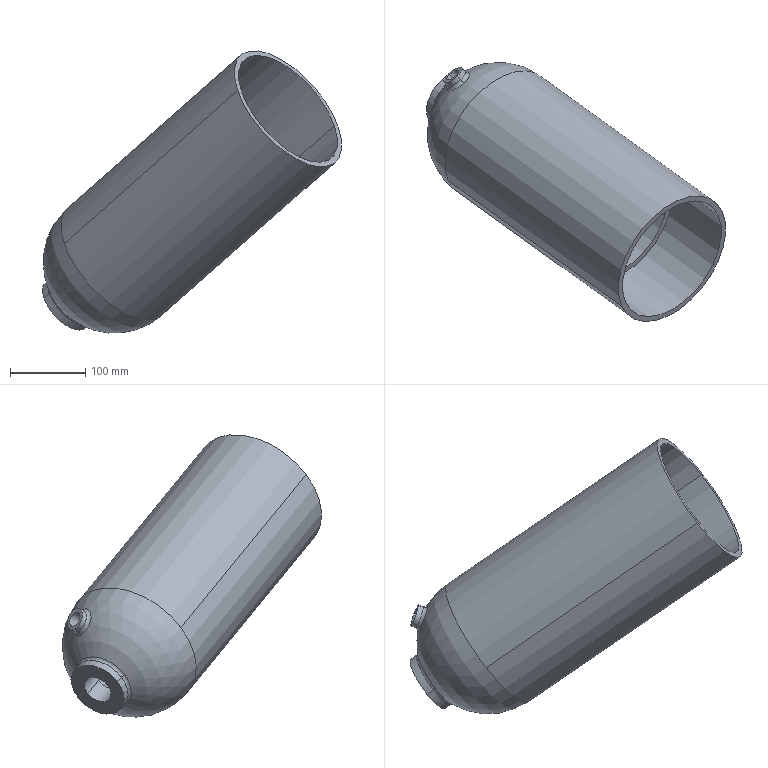Component | SolidWorks | Sleeve-1 | 1 solid | 32 faces | box 398.16 x 345.25 x 375.91 mm | volume 3252942 mm3 | cylinder 18 | torus 6 | plane 6 | sphere 2 | commonest cylinder face diameters 30 x4 81 x2 20 x2 175 x2 40 x2 80 x2 190 x2 160 x2 | material 201.0-T7 Insulated Mold Casting (SS)
STEP:
#1=COLOUR_RGB('',0.7922,0.8196,0.9333);
#2=FILL_AREA_STYLE_COLOUR('',#1);
#3=FILL_AREA_STYLE('',(#2));
#4=SURFACE_STYLE_FILL_AREA(#3);
#5=SURFACE_SIDE_STYLE('',(#4));
#6=SURFACE_STYLE_USAGE(.BOTH.,#5);
#7=PRESENTATION_STYLE_ASSIGNMENT((#6));
#8=CARTESIAN_POINT('',(-9.661,-61.037,0.8353));
#9=VERTEX_POINT('',#8);
#10=CARTESIAN_POINT('',(-11.906,-63.151,1.649));
#11=VERTEX_POINT('',#10);
#12=CARTESIAN_POINT('',(-10.784,-62.094,1.242));
#13=DIRECTION('',(-0.6592,0.4763,-0.5818));
#14=DIRECTION('',(0.704,0.6628,-0.2551));
#15=AXIS2_PLACEMENT_3D('',#12,#13,#14);
#16=CIRCLE('',#15,1.594);
#17=EDGE_CURVE('',#9,#11,#16,.T.);
#18=ORIENTED_EDGE('',*,*,#17,.F.);
#19=CARTESIAN_POINT('',(-9.687,-61.018,0.8122));
#20=VERTEX_POINT('',#19);
#21=CARTESIAN_POINT('',(-9.544,-61.121,0.9382));
#22=DIRECTION('',(-0.6592,0.4763,-0.5818));
#23=VECTOR('',#22,39.37);
#24=LINE('',#21,#23);
#25=EDGE_CURVE('',#9,#20,#24,.T.);
#26=ORIENTED_EDGE('',*,*,#25,.T.);
#27=CARTESIAN_POINT('',(-11.932,-63.132,1.626));
#28=VERTEX_POINT('',#27);
#29=CARTESIAN_POINT('',(-10.81,-62.075,1.219));
#30=DIRECTION('',(0.6592,-0.4763,0.5818));
#31=DIRECTION('',(0.704,0.6628,-0.2551));
#32=AXIS2_PLACEMENT_3D('',#29,#30,#31);
#33=CIRCLE('',#32,1.594);
#34=EDGE_CURVE('',#28,#20,#33,.T.);
#35=ORIENTED_EDGE('',*,*,#34,.F.);
#36=CARTESIAN_POINT('',(-11.79,-63.235,1.752));
#37=DIRECTION('',(-0.6592,0.4763,-0.5818));
#38=VECTOR('',#37,39.37);
#39=LINE('',#36,#38);
#40=EDGE_CURVE('',#11,#28,#39,.T.);
#41=ORIENTED_EDGE('',*,*,#40,.F.);
#42=EDGE_LOOP('',(#18,#26,#35,#41));
#43=FACE_OUTER_BOUND('',#42,.T.);
#44=CARTESIAN_POINT('',(-10.667,-62.178,1.345));
#45=DIRECTION('',(-0.6592,0.4763,-0.5818));
#46=DIRECTION('',(-0.704,-0.6628,0.2551));
#47=AXIS2_PLACEMENT_3D('',#44,#45,#46);
#48=CYLINDRICAL_SURFACE('',#47,1.594);
#49=ADVANCED_FACE('',(#43),#48,.F.);
#50=CARTESIAN_POINT('',(-12.38,-62.912,1.308));
#51=VERTEX_POINT('',#50);
#52=CARTESIAN_POINT('',(-10.01,-60.681,0.4497));
#53=VERTEX_POINT('',#52);
#54=CARTESIAN_POINT('',(-11.195,-61.797,0.879));
#55=DIRECTION('',(0.6592,-0.4763,0.5818));
#56=DIRECTION('',(0.704,0.6628,-0.2551));
#57=AXIS2_PLACEMENT_3D('',#54,#55,#56);
#58=CIRCLE('',#57,1.683);
#59=EDGE_CURVE('',#51,#53,#58,.T.);
#60=ORIENTED_EDGE('',*,*,#59,.F.);
#61=CARTESIAN_POINT('',(-12.419,-62.757,1.178));
#62=VERTEX_POINT('',#61);
#63=CARTESIAN_POINT('',(-12.558,-62.887,1.229));
#64=DIRECTION('',(-0.2641,0.5778,0.7723));
#65=DIRECTION('',(0.,-0.8007,0.599));
#66=AXIS2_PLACEMENT_3D('',#63,#64,#65);
#67=CIRCLE('',#66,0.1969);
#68=EDGE_CURVE('',#51,#62,#67,.T.);
#69=ORIENTED_EDGE('',*,*,#68,.T.);
#70=CARTESIAN_POINT('',(-10.202,-60.669,0.375));
#71=VERTEX_POINT('',#70);
#72=CARTESIAN_POINT('',(-11.311,-61.713,0.7767));
#73=DIRECTION('',(-0.6592,0.4763,-0.5818));
#74=DIRECTION('',(0.704,0.6628,-0.2551));
#75=AXIS2_PLACEMENT_3D('',#72,#73,#74);
#76=CIRCLE('',#75,1.575);
#77=EDGE_CURVE('',#71,#62,#76,.T.);
#78=ORIENTED_EDGE('',*,*,#77,.F.);
#79=CARTESIAN_POINT('',(-10.063,-60.539,0.3248));
#80=DIRECTION('',(0.2641,-0.5778,-0.7723));
#81=DIRECTION('',(0.,0.8007,-0.599));
#82=AXIS2_PLACEMENT_3D('',#79,#80,#81);
#83=CIRCLE('',#82,0.1969);
#84=EDGE_CURVE('',#53,#71,#83,.T.);
#85=ORIENTED_EDGE('',*,*,#84,.F.);
#86=EDGE_LOOP('',(#60,#69,#78,#85));
#87=FACE_OUTER_BOUND('',#86,.T.);
#88=CARTESIAN_POINT('',(-11.311,-61.713,0.7767));
#89=DIRECTION('',(0.6592,-0.4763,0.5818));
#90=DIRECTION('',(0.704,0.6628,-0.2551));
#91=AXIS2_PLACEMENT_3D('',#88,#89,#90);
#92=TOROIDAL_SURFACE('',#91,1.772,0.1969);
#93=ADVANCED_FACE('',(#87),#92,.F.);
#94=CARTESIAN_POINT('',(-10.392,-61.326,4.319));
#95=VERTEX_POINT('',#94);
#96=CARTESIAN_POINT('',(-10.88,-61.219,3.249));
#97=VERTEX_POINT('',#96);
#98=CARTESIAN_POINT('',(-10.636,-61.272,3.784));
#99=DIRECTION('',(0.5773,-0.7433,-0.3379));
#100=DIRECTION('',(-0.4136,0.09066,-0.906));
#101=AXIS2_PLACEMENT_3D('',#98,#99,#100);
#102=CIRCLE('',#101,0.5906);
#103=EDGE_CURVE('',#95,#97,#102,.T.);
#104=ORIENTED_EDGE('',*,*,#103,.F.);
#105=CARTESIAN_POINT('',(-10.398,-61.207,4.609));
#106=VERTEX_POINT('',#105);
#107=CARTESIAN_POINT('',(-10.31,-61.344,4.497));
#108=DIRECTION('',(0.704,0.6628,-0.2551));
#109=DIRECTION('',(-0.6855,0.7281,0.));
#110=AXIS2_PLACEMENT_3D('',#107,#108,#109);
#111=CIRCLE('',#110,0.1969);
#112=EDGE_CURVE('',#95,#106,#111,.T.);
#113=ORIENTED_EDGE('',*,*,#112,.T.);
#114=CARTESIAN_POINT('',(-11.093,-61.055,3.087));
#115=VERTEX_POINT('',#114);
#116=CARTESIAN_POINT('',(-10.745,-61.131,3.848));
#117=DIRECTION('',(-0.5773,0.7433,0.3379));
#118=DIRECTION('',(-0.4136,0.09066,-0.906));
#119=AXIS2_PLACEMENT_3D('',#116,#117,#118);
#120=CIRCLE('',#119,0.8399);
#121=EDGE_CURVE('',#115,#106,#120,.T.);
#122=ORIENTED_EDGE('',*,*,#121,.F.);
#123=CARTESIAN_POINT('',(-10.962,-61.201,3.071));
#124=DIRECTION('',(-0.704,-0.6628,0.2551));
#125=DIRECTION('',(0.6855,-0.7281,0.));
#126=AXIS2_PLACEMENT_3D('',#123,#124,#125);
#127=CIRCLE('',#126,0.1969);
#128=EDGE_CURVE('',#97,#115,#127,.T.);
#129=ORIENTED_EDGE('',*,*,#128,.F.);
#130=EDGE_LOOP('',(#104,#113,#122,#129));
#131=FACE_OUTER_BOUND('',#130,.T.);
#132=CARTESIAN_POINT('',(-10.636,-61.272,3.784));
#133=DIRECTION('',(0.5773,-0.7433,-0.3379));
#134=DIRECTION('',(-0.4136,0.09066,-0.906));
#135=AXIS2_PLACEMENT_3D('',#132,#133,#134);
#136=TOROIDAL_SURFACE('',#135,0.7874,0.1969);
#137=ADVANCED_FACE('',(#131),#136,.F.);
#138=CARTESIAN_POINT('',(-10.799,-60.732,4.738));
#139=VERTEX_POINT('',#138);
#140=CARTESIAN_POINT('',(-11.418,-60.596,3.383));
#141=VERTEX_POINT('',#140);
#142=CARTESIAN_POINT('',(-11.109,-60.664,4.061));
#143=DIRECTION('',(0.5773,-0.7433,-0.3379));
#144=DIRECTION('',(-0.4136,0.09066,-0.906));
#145=AXIS2_PLACEMENT_3D('',#142,#143,#144);
#146=CIRCLE('',#145,0.748);
#147=EDGE_CURVE('',#139,#141,#146,.T.);
#148=ORIENTED_EDGE('',*,*,#147,.F.);
#149=CARTESIAN_POINT('',(-10.976,-60.574,4.661));
#150=VERTEX_POINT('',#149);
#151=CARTESIAN_POINT('',(-10.894,-60.592,4.839));
#152=DIRECTION('',(0.704,0.6628,-0.2551));
#153=DIRECTION('',(-0.6855,0.7281,0.));
#154=AXIS2_PLACEMENT_3D('',#151,#152,#153);
#155=CIRCLE('',#154,0.1969);
#156=EDGE_CURVE('',#139,#150,#155,.T.);
#157=ORIENTED_EDGE('',*,*,#156,.T.);
#158=CARTESIAN_POINT('',(-11.464,-60.467,3.591));
#159=VERTEX_POINT('',#158);
#160=CARTESIAN_POINT('',(-11.22,-60.52,4.126));
#161=DIRECTION('',(-0.5773,0.7433,0.3379));
#162=DIRECTION('',(-0.4136,0.09066,-0.906));
#163=AXIS2_PLACEMENT_3D('',#160,#161,#162);
#164=CIRCLE('',#163,0.5906);
#165=EDGE_CURVE('',#159,#150,#164,.T.);
#166=ORIENTED_EDGE('',*,*,#165,.F.);
#167=CARTESIAN_POINT('',(-11.546,-60.449,3.413));
#168=DIRECTION('',(-0.704,-0.6628,0.2551));
#169=DIRECTION('',(0.6855,-0.7281,0.));
#170=AXIS2_PLACEMENT_3D('',#167,#168,#169);
#171=CIRCLE('',#170,0.1969);
#172=EDGE_CURVE('',#141,#159,#171,.T.);
#173=ORIENTED_EDGE('',*,*,#172,.F.);
#174=EDGE_LOOP('',(#148,#157,#166,#173));
#175=FACE_OUTER_BOUND('',#174,.T.);
#176=CARTESIAN_POINT('',(-11.22,-60.52,4.126));
#177=DIRECTION('',(0.5773,-0.7433,-0.3379));
#178=DIRECTION('',(-0.4136,0.09066,-0.906));
#179=AXIS2_PLACEMENT_3D('',#176,#177,#178);
#180=TOROIDAL_SURFACE('',#179,0.7874,0.1969);
#181=ADVANCED_FACE('',(#175),#180,.F.);
#182=CARTESIAN_POINT('',(-11.544,-60.277,3.864));
#183=VERTEX_POINT('',#182);
#184=CARTESIAN_POINT('',(-11.219,-60.348,4.577));
#185=VERTEX_POINT('',#184);
#186=CARTESIAN_POINT('',(-11.381,-60.313,4.22));
#187=DIRECTION('',(-0.5773,0.7433,0.3379));
#188=DIRECTION('',(0.4136,-0.09066,0.906));
#189=AXIS2_PLACEMENT_3D('',#186,#187,#188);
#190=CIRCLE('',#189,0.3937);
#191=EDGE_CURVE('',#183,#185,#190,.T.);
#192=ORIENTED_EDGE('',*,*,#191,.T.);
#193=CARTESIAN_POINT('',(-10.423,-61.373,4.111));
#194=VERTEX_POINT('',#193);
#195=CARTESIAN_POINT('',(-11.219,-60.348,4.577));
#196=DIRECTION('',(0.5773,-0.7433,-0.3379));
#197=VECTOR('',#196,39.37);
#198=LINE('',#195,#197);
#199=EDGE_CURVE('',#185,#194,#198,.T.);
#200=ORIENTED_EDGE('',*,*,#199,.T.);
#201=CARTESIAN_POINT('',(-10.749,-61.301,3.398));
#202=VERTEX_POINT('',#201);
#203=CARTESIAN_POINT('',(-10.586,-61.337,3.755));
#204=DIRECTION('',(-0.5773,0.7433,0.3379));
#205=DIRECTION('',(0.4136,-0.09066,0.906));
#206=AXIS2_PLACEMENT_3D('',#203,#204,#205);
#207=CIRCLE('',#206,0.3937);
#208=EDGE_CURVE('',#202,#194,#207,.T.);
#209=ORIENTED_EDGE('',*,*,#208,.F.);
#210=CARTESIAN_POINT('',(-11.544,-60.277,3.864));
#211=DIRECTION('',(0.5773,-0.7433,-0.3379));
#212=VECTOR('',#211,39.37);
#213=LINE('',#210,#212);
#214=EDGE_CURVE('',#183,#202,#213,.T.);
#215=ORIENTED_EDGE('',*,*,#214,.F.);
#216=EDGE_LOOP('',(#192,#200,#209,#215));
#217=FACE_OUTER_BOUND('',#216,.T.);
#218=CARTESIAN_POINT('',(-11.381,-60.313,4.22));
#219=DIRECTION('',(0.5773,-0.7433,-0.3379));
#220=DIRECTION('',(-0.4136,0.09066,-0.906));
#221=AXIS2_PLACEMENT_3D('',#218,#219,#220);
#222=CYLINDRICAL_SURFACE('',#221,0.3937);
#223=ADVANCED_FACE('',(#217),#222,.F.);
#224=CARTESIAN_POINT('',(-11.22,-60.52,4.126));
#225=DIRECTION('',(-0.5773,0.7433,0.3379));
#226=DIRECTION('',(-0.4136,0.09066,-0.906));
#227=AXIS2_PLACEMENT_3D('',#224,#225,#226);
#228=CIRCLE('',#227,0.5906);
#229=EDGE_CURVE('',#150,#159,#228,.T.);
#230=ORIENTED_EDGE('',*,*,#229,.T.);
#231=CARTESIAN_POINT('',(-11.626,-60.259,3.685));
#232=VERTEX_POINT('',#231);
#233=CARTESIAN_POINT('',(-10.83,-61.283,3.22));
#234=DIRECTION('',(-0.5773,0.7433,0.3379));
#235=VECTOR('',#234,39.37);
#236=LINE('',#233,#235);
#237=EDGE_CURVE('',#159,#232,#236,.T.);
#238=ORIENTED_EDGE('',*,*,#237,.T.);
#239=CARTESIAN_POINT('',(-11.137,-60.366,4.755));
#240=VERTEX_POINT('',#239);
#241=CARTESIAN_POINT('',(-11.381,-60.313,4.22));
#242=DIRECTION('',(-0.5773,0.7433,0.3379));
#243=DIRECTION('',(0.4136,-0.09066,0.906));
#244=AXIS2_PLACEMENT_3D('',#241,#242,#243);
#245=CIRCLE('',#244,0.5906);
#246=EDGE_CURVE('',#240,#232,#245,.T.);
#247=ORIENTED_EDGE('',*,*,#246,.F.);
#248=CARTESIAN_POINT('',(-10.342,-61.39,4.29));
#249=DIRECTION('',(-0.5773,0.7433,0.3379));
#250=VECTOR('',#249,39.37);
#251=LINE('',#248,#250);
#252=EDGE_CURVE('',#150,#240,#251,.T.);
#253=ORIENTED_EDGE('',*,*,#252,.F.);
#254=EDGE_LOOP('',(#230,#238,#247,#253));
#255=FACE_OUTER_BOUND('',#254,.T.);
#256=CARTESIAN_POINT('',(-10.586,-61.337,3.755));
#257=DIRECTION('',(-0.5773,0.7433,0.3379));
#258=DIRECTION('',(0.4136,-0.09066,0.906));
#259=AXIS2_PLACEMENT_3D('',#256,#257,#258);
#260=CYLINDRICAL_SURFACE('',#259,0.5906);
#261=ADVANCED_FACE('',(#255),#260,.T.);
#262=CARTESIAN_POINT('',(-10.342,-61.39,4.29));
#263=VERTEX_POINT('',#262);
#264=CARTESIAN_POINT('',(-10.83,-61.283,3.22));
#265=VERTEX_POINT('',#264);
#266=CARTESIAN_POINT('',(-10.586,-61.337,3.755));
#267=DIRECTION('',(-0.5773,0.7433,0.3379));
#268=DIRECTION('',(0.4136,-0.09066,0.906));
#269=AXIS2_PLACEMENT_3D('',#266,#267,#268);
#270=CIRCLE('',#269,0.5906);
#271=EDGE_CURVE('',#263,#265,#270,.T.);
#272=ORIENTED_EDGE('',*,*,#271,.T.);
#273=CARTESIAN_POINT('',(-10.83,-61.283,3.22));
#274=DIRECTION('',(-0.5773,0.7433,0.3379));
#275=VECTOR('',#274,39.37);
#276=LINE('',#273,#275);
#277=EDGE_CURVE('',#265,#97,#276,.T.);
#278=ORIENTED_EDGE('',*,*,#277,.T.);
#279=CARTESIAN_POINT('',(-10.636,-61.272,3.784));
#280=DIRECTION('',(0.5773,-0.7433,-0.3379));
#281=DIRECTION('',(-0.4136,0.09066,-0.906));
#282=AXIS2_PLACEMENT_3D('',#279,#280,#281);
#283=CIRCLE('',#282,0.5906);
#284=EDGE_CURVE('',#97,#95,#283,.T.);
#285=ORIENTED_EDGE('',*,*,#284,.T.);
#286=CARTESIAN_POINT('',(-10.342,-61.39,4.29));
#287=DIRECTION('',(-0.5773,0.7433,0.3379));
#288=VECTOR('',#287,39.37);
#289=LINE('',#286,#288);
#290=EDGE_CURVE('',#263,#95,#289,.T.);
#291=ORIENTED_EDGE('',*,*,#290,.F.);
#292=EDGE_LOOP('',(#272,#278,#285,#291));
#293=FACE_OUTER_BOUND('',#292,.T.);
#294=CARTESIAN_POINT('',(-10.586,-61.337,3.755));
#295=DIRECTION('',(-0.5773,0.7433,0.3379));
#296=DIRECTION('',(0.4136,-0.09066,0.906));
#297=AXIS2_PLACEMENT_3D('',#294,#295,#296);
#298=CYLINDRICAL_SURFACE('',#297,0.5906);
#299=ADVANCED_FACE('',(#293),#298,.T.);
#300=CARTESIAN_POINT('',(-2.334,-72.234,11.718));
#301=VERTEX_POINT('',#300);
#302=CARTESIAN_POINT('',(2.516,-67.668,9.961));
#303=VERTEX_POINT('',#302);
#304=CARTESIAN_POINT('',(0.09081,-69.951,10.84));
#305=DIRECTION('',(0.6592,-0.4763,0.5818));
#306=DIRECTION('',(0.704,0.6628,-0.2551));
#307=AXIS2_PLACEMENT_3D('',#304,#305,#306);
#308=CIRCLE('',#307,3.445);
#309=EDGE_CURVE('',#301,#303,#308,.T.);
#310=ORIENTED_EDGE('',*,*,#309,.T.);
#311=CARTESIAN_POINT('',(-0.07926,-65.793,7.67));
#312=VERTEX_POINT('',#311);
#313=CARTESIAN_POINT('',(2.516,-67.668,9.961));
#314=DIRECTION('',(-0.6592,0.4763,-0.5818));
#315=VECTOR('',#314,39.37);
#316=LINE('',#313,#315);
#317=EDGE_CURVE('',#303,#312,#316,.T.);
#318=ORIENTED_EDGE('',*,*,#317,.T.);
#319=CARTESIAN_POINT('',(-4.93,-70.359,9.428));
#320=VERTEX_POINT('',#319);
#321=CARTESIAN_POINT('',(-2.505,-68.076,8.549));
#322=DIRECTION('',(0.6592,-0.4763,0.5818));
#323=DIRECTION('',(0.704,0.6628,-0.2551));
#324=AXIS2_PLACEMENT_3D('',#321,#322,#323);
#325=CIRCLE('',#324,3.445);
#326=EDGE_CURVE('',#320,#312,#325,.T.);
#327=ORIENTED_EDGE('',*,*,#326,.F.);
#328=CARTESIAN_POINT('',(-2.334,-72.234,11.718));
#329=DIRECTION('',(-0.6592,0.4763,-0.5818));
#330=VECTOR('',#329,39.37);
#331=LINE('',#328,#330);
#332=EDGE_CURVE('',#301,#320,#331,.T.);
#333=ORIENTED_EDGE('',*,*,#332,.F.);
#334=EDGE_LOOP('',(#310,#318,#327,#333));
#335=FACE_OUTER_BOUND('',#334,.T.);
#336=CARTESIAN_POINT('',(0.09081,-69.951,10.84));
#337=DIRECTION('',(-0.6592,0.4763,-0.5818));
#338=DIRECTION('',(-0.704,-0.6628,0.2551));
#339=AXIS2_PLACEMENT_3D('',#336,#337,#338);
#340=CYLINDRICAL_SURFACE('',#339,3.445);
#341=ADVANCED_FACE('',(#335),#340,.F.);
#342=CARTESIAN_POINT('',(-11.364,-62.597,1.42));
#343=VERTEX_POINT('',#342);
#344=CARTESIAN_POINT('',(-10.255,-61.553,1.018));
#345=VERTEX_POINT('',#344);
#346=CARTESIAN_POINT('',(-10.81,-62.075,1.219));
#347=DIRECTION('',(0.6592,-0.4763,0.5818));
#348=DIRECTION('',(0.704,0.6628,-0.2551));
#349=AXIS2_PLACEMENT_3D('',#346,#347,#348);
#350=CIRCLE('',#349,0.7874);
#351=EDGE_CURVE('',#343,#345,#350,.T.);
#352=ORIENTED_EDGE('',*,*,#351,.T.);
#353=CARTESIAN_POINT('',(-11.034,-60.99,0.3308));
#354=VERTEX_POINT('',#353);
#355=CARTESIAN_POINT('',(-10.385,-61.459,0.9035));
#356=DIRECTION('',(-0.6592,0.4763,-0.5818));
#357=VECTOR('',#356,39.37);
#358=LINE('',#355,#357);
#359=EDGE_CURVE('',#345,#354,#358,.T.);
#360=ORIENTED_EDGE('',*,*,#359,.T.);
#361=CARTESIAN_POINT('',(-12.143,-62.034,0.7325));
#362=VERTEX_POINT('',#361);
#363=CARTESIAN_POINT('',(-11.588,-61.512,0.5317));
#364=DIRECTION('',(0.6592,-0.4763,0.5818));
#365=DIRECTION('',(0.704,0.6628,-0.2551));
#366=AXIS2_PLACEMENT_3D('',#363,#364,#365);
#367=CIRCLE('',#366,0.7874);
#368=EDGE_CURVE('',#362,#354,#367,.T.);
#369=ORIENTED_EDGE('',*,*,#368,.F.);
#370=CARTESIAN_POINT('',(-11.494,-62.503,1.305));
#371=DIRECTION('',(-0.6592,0.4763,-0.5818));
#372=VECTOR('',#371,39.37);
#373=LINE('',#370,#372);
#374=EDGE_CURVE('',#343,#362,#373,.T.);
#375=ORIENTED_EDGE('',*,*,#374,.F.);
#376=EDGE_LOOP('',(#352,#360,#369,#375));
#377=FACE_OUTER_BOUND('',#376,.T.);
#378=CARTESIAN_POINT('',(-10.939,-61.981,1.104));
#379=DIRECTION('',(-0.6592,0.4763,-0.5818));
#380=DIRECTION('',(-0.704,-0.6628,0.2551));
#381=AXIS2_PLACEMENT_3D('',#378,#379,#380);
#382=CYLINDRICAL_SURFACE('',#381,0.7874);
#383=ADVANCED_FACE('',(#377),#382,.F.);
#384=CARTESIAN_POINT('',(-11.311,-61.713,0.7767));
#385=DIRECTION('',(-0.6592,0.4763,-0.5818));
#386=DIRECTION('',(0.704,0.6628,-0.2551));
#387=AXIS2_PLACEMENT_3D('',#384,#385,#386);
#388=CIRCLE('',#387,1.575);
#389=EDGE_CURVE('',#62,#71,#388,.T.);
#390=ORIENTED_EDGE('',*,*,#389,.T.);
#391=CARTESIAN_POINT('',(-10.48,-60.469,0.13));
#392=VERTEX_POINT('',#391);
#393=CARTESIAN_POINT('',(-9.701,-61.031,0.8172));
#394=DIRECTION('',(-0.6592,0.4763,-0.5818));
#395=VECTOR('',#394,39.37);
#396=LINE('',#393,#395);
#397=EDGE_CURVE('',#71,#392,#396,.T.);
#398=ORIENTED_EDGE('',*,*,#397,.T.);
#399=CARTESIAN_POINT('',(-12.697,-62.556,0.9333));
#400=VERTEX_POINT('',#399);
#401=CARTESIAN_POINT('',(-11.588,-61.512,0.5317));
#402=DIRECTION('',(0.6592,-0.4763,0.5818));
#403=DIRECTION('',(0.704,0.6628,-0.2551));
#404=AXIS2_PLACEMENT_3D('',#401,#402,#403);
#405=CIRCLE('',#404,1.575);
#406=EDGE_CURVE('',#392,#400,#405,.T.);
#407=ORIENTED_EDGE('',*,*,#406,.T.);
#408=CARTESIAN_POINT('',(-11.918,-63.119,1.621));
#409=DIRECTION('',(-0.6592,0.4763,-0.5818));
#410=VECTOR('',#409,39.37);
#411=LINE('',#408,#410);
#412=EDGE_CURVE('',#62,#400,#411,.T.);
#413=ORIENTED_EDGE('',*,*,#412,.F.);
#414=EDGE_LOOP('',(#390,#398,#407,#413));
#415=FACE_OUTER_BOUND('',#414,.T.);
#416=CARTESIAN_POINT('',(-10.81,-62.075,1.219));
#417=DIRECTION('',(-0.6592,0.4763,-0.5818));
#418=DIRECTION('',(-0.704,-0.6628,0.2551));
#419=AXIS2_PLACEMENT_3D('',#416,#417,#418);
#420=CYLINDRICAL_SURFACE('',#419,1.575);
#421=ADVANCED_FACE('',(#415),#420,.T.);
#422=CARTESIAN_POINT('',(2.724,-67.472,9.886));
#423=VERTEX_POINT('',#422);
#424=CARTESIAN_POINT('',(-2.542,-72.43,11.794));
#425=VERTEX_POINT('',#424);
#426=CARTESIAN_POINT('',(0.09081,-69.951,10.84));
#427=DIRECTION('',(0.6592,-0.4763,0.5818));
#428=DIRECTION('',(0.704,0.6628,-0.2551));
#429=AXIS2_PLACEMENT_3D('',#426,#427,#428);
#430=CIRCLE('',#429,3.74);
#431=EDGE_CURVE('',#423,#425,#430,.T.);
#432=ORIENTED_EDGE('',*,*,#431,.F.);
#433=CARTESIAN_POINT('',(-6.36,-60.909,1.868));
#434=VERTEX_POINT('',#433);
#435=CARTESIAN_POINT('',(2.724,-67.472,9.886));
#436=DIRECTION('',(-0.6592,0.4763,-0.5818));
#437=VECTOR('',#436,39.37);
#438=LINE('',#435,#437);
#439=EDGE_CURVE('',#423,#434,#438,.T.);
#440=ORIENTED_EDGE('',*,*,#439,.T.);
#441=CARTESIAN_POINT('',(-11.626,-65.867,3.776));
#442=VERTEX_POINT('',#441);
#443=CARTESIAN_POINT('',(-8.993,-63.388,2.822));
#444=DIRECTION('',(0.6592,-0.4763,0.5818));
#445=DIRECTION('',(0.2641,-0.5778,-0.7723));
#446=AXIS2_PLACEMENT_3D('',#443,#444,#445);
#447=CIRCLE('',#446,3.74);
#448=EDGE_CURVE('',#434,#442,#447,.T.);
#449=ORIENTED_EDGE('',*,*,#448,.T.);
#450=CARTESIAN_POINT('',(-2.542,-72.43,11.794));
#451=DIRECTION('',(-0.6592,0.4763,-0.5818));
#452=VECTOR('',#451,39.37);
#453=LINE('',#450,#452);
#454=EDGE_CURVE('',#425,#442,#453,.T.);
#455=ORIENTED_EDGE('',*,*,#454,.F.);
#456=EDGE_LOOP('',(#432,#440,#449,#455));
#457=FACE_OUTER_BOUND('',#456,.T.);
#458=CARTESIAN_POINT('',(0.09081,-69.951,10.84));
#459=DIRECTION('',(-0.6592,0.4763,-0.5818));
#460=DIRECTION('',(-0.704,-0.6628,0.2551));
#461=AXIS2_PLACEMENT_3D('',#458,#459,#460);
#462=CYLINDRICAL_SURFACE('',#461,3.74);
#463=ADVANCED_FACE('',(#457),#462,.T.);
#464=CARTESIAN_POINT('',(-4.722,-70.163,9.352));
#465=VERTEX_POINT('',#464);
#466=CARTESIAN_POINT('',(-0.2871,-65.988,7.746));
#467=VERTEX_POINT('',#466);
#468=CARTESIAN_POINT('',(-2.505,-68.076,8.549));
#469=DIRECTION('',(0.6592,-0.4763,0.5818));
#470=DIRECTION('',(0.704,0.6628,-0.2551));
#471=AXIS2_PLACEMENT_3D('',#468,#469,#470);
#472=CIRCLE('',#471,3.15);
#473=EDGE_CURVE('',#465,#467,#472,.T.);
#474=ORIENTED_EDGE('',*,*,#473,.T.);
#475=CARTESIAN_POINT('',(-6.776,-61.3,2.019));
#476=VERTEX_POINT('',#475);
#477=CARTESIAN_POINT('',(2.308,-67.864,10.036));
#478=DIRECTION('',(-0.6592,0.4763,-0.5818));
#479=VECTOR('',#478,39.37);
#480=LINE('',#477,#479);
#481=EDGE_CURVE('',#467,#476,#480,.T.);
#482=ORIENTED_EDGE('',*,*,#481,.T.);
#483=CARTESIAN_POINT('',(-11.21,-65.475,3.626));
#484=VERTEX_POINT('',#483);
#485=CARTESIAN_POINT('',(-8.993,-63.388,2.822));
#486=DIRECTION('',(0.6592,-0.4763,0.5818));
#487=DIRECTION('',(0.704,0.6628,-0.2551));
#488=AXIS2_PLACEMENT_3D('',#485,#486,#487);
#489=CIRCLE('',#488,3.15);
#490=EDGE_CURVE('',#484,#476,#489,.T.);
#491=ORIENTED_EDGE('',*,*,#490,.F.);
#492=CARTESIAN_POINT('',(-2.127,-72.039,11.643));
#493=DIRECTION('',(-0.6592,0.4763,-0.5818));
#494=VECTOR('',#493,39.37);
#495=LINE('',#492,#494);
#496=EDGE_CURVE('',#465,#484,#495,.T.);
#497=ORIENTED_EDGE('',*,*,#496,.F.);
#498=EDGE_LOOP('',(#474,#482,#491,#497));
#499=FACE_OUTER_BOUND('',#498,.T.);
#500=CARTESIAN_POINT('',(0.09081,-69.951,10.84));
#501=DIRECTION('',(-0.6592,0.4763,-0.5818));
#502=DIRECTION('',(-0.704,-0.6628,0.2551));
#503=AXIS2_PLACEMENT_3D('',#500,#501,#502);
#504=CYLINDRICAL_SURFACE('',#503,3.15);
#505=ADVANCED_FACE('',(#499),#504,.F.);
#506=ORIENTED_EDGE('',*,*,#490,.T.);
#507=CARTESIAN_POINT('',(-8.993,-63.388,2.822));
#508=DIRECTION('',(0.6592,-0.4763,0.5818));
#509=DIRECTION('',(0.704,0.6628,-0.2551));
#510=AXIS2_PLACEMENT_3D('',#507,#508,#509);
#511=CIRCLE('',#510,3.15);
#512=EDGE_CURVE('',#476,#484,#511,.T.);
#513=ORIENTED_EDGE('',*,*,#512,.T.);
#514=EDGE_LOOP('',(#506,#513));
#515=FACE_OUTER_BOUND('',#514,.T.);
#516=ORIENTED_EDGE('',*,*,#121,.T.);
#517=CARTESIAN_POINT('',(-10.745,-61.131,3.848));
#518=DIRECTION('',(-0.5773,0.7433,0.3379));
#519=DIRECTION('',(-0.4136,0.09066,-0.906));
#520=AXIS2_PLACEMENT_3D('',#517,#518,#519);
#521=CIRCLE('',#520,0.8399);
#522=EDGE_CURVE('',#106,#115,#521,.T.);
#523=ORIENTED_EDGE('',*,*,#522,.T.);
#524=EDGE_LOOP('',(#516,#523));
#525=FACE_BOUND('',#524,.T.);
#526=CARTESIAN_POINT('',(-10.784,-62.094,1.242));
#527=DIRECTION('',(-0.6592,0.4763,-0.5818));
#528=DIRECTION('',(0.704,0.6628,-0.2551));
#529=AXIS2_PLACEMENT_3D('',#526,#527,#528);
#530=CIRCLE('',#529,1.594);
#531=EDGE_CURVE('',#11,#9,#530,.T.);
#532=ORIENTED_EDGE('',*,*,#531,.T.);
#533=ORIENTED_EDGE('',*,*,#17,.T.);
#534=EDGE_LOOP('',(#532,#533));
#535=FACE_BOUND('',#534,.T.);
#536=CARTESIAN_POINT('',(-8.993,-63.388,2.822));
#537=DIRECTION('',(0.6592,-0.4763,0.5818));
#538=DIRECTION('',(0.704,0.6628,-0.2551));
#539=AXIS2_PLACEMENT_3D('',#536,#537,#538);
#540=SPHERICAL_SURFACE('',#539,3.15);
#541=ADVANCED_FACE('',(#515,#525,#535),#540,.F.);
#542=ORIENTED_EDGE('',*,*,#481,.F.);
#543=CARTESIAN_POINT('',(-2.505,-68.076,8.549));
#544=DIRECTION('',(0.6592,-0.4763,0.5818));
#545=DIRECTION('',(0.704,0.6628,-0.2551));
#546=AXIS2_PLACEMENT_3D('',#543,#544,#545);
#547=CIRCLE('',#546,3.15);
#548=EDGE_CURVE('',#467,#465,#547,.T.);
#549=ORIENTED_EDGE('',*,*,#548,.T.);
#550=ORIENTED_EDGE('',*,*,#496,.T.);
#551=ORIENTED_EDGE('',*,*,#512,.F.);
#552=EDGE_LOOP('',(#542,#549,#550,#551));
#553=FACE_OUTER_BOUND('',#552,.T.);
#554=CARTESIAN_POINT('',(0.09081,-69.951,10.84));
#555=DIRECTION('',(-0.6592,0.4763,-0.5818));
#556=DIRECTION('',(-0.704,-0.6628,0.2551));
#557=AXIS2_PLACEMENT_3D('',#554,#555,#556);
#558=CYLINDRICAL_SURFACE('',#557,3.15);
#559=ADVANCED_FACE('',(#553),#558,.F.);
#560=CARTESIAN_POINT('',(-11.195,-61.797,0.879));
#561=DIRECTION('',(0.6592,-0.4763,0.5818));
#562=DIRECTION('',(0.704,0.6628,-0.2551));
#563=AXIS2_PLACEMENT_3D('',#560,#561,#562);
#564=CIRCLE('',#563,1.683);
#565=EDGE_CURVE('',#53,#51,#564,.T.);
#566=ORIENTED_EDGE('',*,*,#565,.T.);
#567=ORIENTED_EDGE('',*,*,#59,.T.);
#568=EDGE_LOOP('',(#566,#567));
#569=FACE_BOUND('',#568,.T.);
#570=CARTESIAN_POINT('',(-11.109,-60.664,4.061));
#571=DIRECTION('',(0.5773,-0.7433,-0.3379));
#572=DIRECTION('',(-0.4136,0.09066,-0.906));
#573=AXIS2_PLACEMENT_3D('',#570,#571,#572);
#574=CIRCLE('',#573,0.748);
#575=EDGE_CURVE('',#141,#139,#574,.T.);
#576=ORIENTED_EDGE('',*,*,#575,.T.);
#577=ORIENTED_EDGE('',*,*,#147,.T.);
#578=EDGE_LOOP('',(#576,#577));
#579=FACE_BOUND('',#578,.T.);
#580=CARTESIAN_POINT('',(-8.993,-63.388,2.822));
#581=DIRECTION('',(0.6592,-0.4763,0.5818));
#582=DIRECTION('',(0.2641,-0.5778,-0.7723));
#583=AXIS2_PLACEMENT_3D('',#580,#581,#582);
#584=CIRCLE('',#583,3.74);
#585=EDGE_CURVE('',#442,#434,#584,.T.);
#586=ORIENTED_EDGE('',*,*,#585,.F.);
#587=ORIENTED_EDGE('',*,*,#448,.F.);
#588=EDGE_LOOP('',(#586,#587));
#589=FACE_OUTER_BOUND('',#588,.T.);
#590=CARTESIAN_POINT('',(-8.993,-63.388,2.822));
#591=DIRECTION('',(0.6592,-0.4763,0.5818));
#592=DIRECTION('',(0.704,0.6628,-0.2551));
#593=AXIS2_PLACEMENT_3D('',#590,#591,#592);
#594=SPHERICAL_SURFACE('',#593,3.74);
#595=ADVANCED_FACE('',(#569,#579,#589),#594,.T.);
#596=ORIENTED_EDGE('',*,*,#309,.F.);
#597=CARTESIAN_POINT('',(0.09081,-69.951,10.84));
#598=DIRECTION('',(0.6592,-0.4763,0.5818));
#599=DIRECTION('',(0.704,0.6628,-0.2551));
#600=AXIS2_PLACEMENT_3D('',#597,#598,#599);
#601=CIRCLE('',#600,3.445);
#602=EDGE_CURVE('',#303,#301,#601,.T.);
#603=ORIENTED_EDGE('',*,*,#602,.F.);
#604=EDGE_LOOP('',(#596,#603));
#605=FACE_BOUND('',#604,.T.);
#606=CARTESIAN_POINT('',(0.09081,-69.951,10.84));
#607=DIRECTION('',(0.6592,-0.4763,0.5818));
#608=DIRECTION('',(0.704,0.6628,-0.2551));
#609=AXIS2_PLACEMENT_3D('',#606,#607,#608);
#610=CIRCLE('',#609,3.74);
#611=EDGE_CURVE('',#425,#423,#610,.T.);
#612=ORIENTED_EDGE('',*,*,#611,.T.);
#613=ORIENTED_EDGE('',*,*,#431,.T.);
#614=EDGE_LOOP('',(#612,#613));
#615=FACE_OUTER_BOUND('',#614,.T.);
#616=CARTESIAN_POINT('',(0.09081,-69.951,10.84));
#617=DIRECTION('',(0.6592,-0.4763,0.5818));
#618=DIRECTION('',(0.704,0.6628,-0.2551));
#619=AXIS2_PLACEMENT_3D('',#616,#617,#618);
#620=PLANE('',#619);
#621=ADVANCED_FACE('',(#605,#615),#620,.T.);
#622=ORIENTED_EDGE('',*,*,#439,.F.);
#623=ORIENTED_EDGE('',*,*,#611,.F.);
#624=ORIENTED_EDGE('',*,*,#454,.T.);
#625=ORIENTED_EDGE('',*,*,#585,.T.);
#626=EDGE_LOOP('',(#622,#623,#624,#625));
#627=FACE_OUTER_BOUND('',#626,.T.);
#628=CARTESIAN_POINT('',(0.09081,-69.951,10.84));
#629=DIRECTION('',(-0.6592,0.4763,-0.5818));
#630=DIRECTION('',(-0.704,-0.6628,0.2551));
#631=AXIS2_PLACEMENT_3D('',#628,#629,#630);
#632=CYLINDRICAL_SURFACE('',#631,3.74);
#633=ADVANCED_FACE('',(#627),#632,.T.);
#634=CARTESIAN_POINT('',(-11.588,-61.512,0.5317));
#635=DIRECTION('',(0.6592,-0.4763,0.5818));
#636=DIRECTION('',(0.704,0.6628,-0.2551));
#637=AXIS2_PLACEMENT_3D('',#634,#635,#636);
#638=CIRCLE('',#637,1.575);
#639=EDGE_CURVE('',#400,#392,#638,.T.);
#640=ORIENTED_EDGE('',*,*,#639,.F.);
#641=ORIENTED_EDGE('',*,*,#406,.F.);
#642=EDGE_LOOP('',(#640,#641));
#643=FACE_OUTER_BOUND('',#642,.T.);
#644=ORIENTED_EDGE('',*,*,#368,.T.);
#645=CARTESIAN_POINT('',(-11.588,-61.512,0.5317));
#646=DIRECTION('',(0.6592,-0.4763,0.5818));
#647=DIRECTION('',(0.704,0.6628,-0.2551));
#648=AXIS2_PLACEMENT_3D('',#645,#646,#647);
#649=CIRCLE('',#648,0.7874);
#650=EDGE_CURVE('',#354,#362,#649,.T.);
#651=ORIENTED_EDGE('',*,*,#650,.T.);
#652=EDGE_LOOP('',(#644,#651));
#653=FACE_BOUND('',#652,.T.);
#654=CARTESIAN_POINT('',(-11.588,-61.512,0.5317));
#655=DIRECTION('',(0.6592,-0.4763,0.5818));
#656=DIRECTION('',(0.704,0.6628,-0.2551));
#657=AXIS2_PLACEMENT_3D('',#654,#655,#656);
#658=PLANE('',#657);
#659=ADVANCED_FACE('',(#643,#653),#658,.F.);
#660=ORIENTED_EDGE('',*,*,#397,.F.);
#661=ORIENTED_EDGE('',*,*,#77,.T.);
#662=ORIENTED_EDGE('',*,*,#412,.T.);
#663=ORIENTED_EDGE('',*,*,#639,.T.);
#664=EDGE_LOOP('',(#660,#661,#662,#663));
#665=FACE_OUTER_BOUND('',#664,.T.);
#666=CARTESIAN_POINT('',(-10.81,-62.075,1.219));
#667=DIRECTION('',(-0.6592,0.4763,-0.5818));
#668=DIRECTION('',(-0.704,-0.6628,0.2551));
#669=AXIS2_PLACEMENT_3D('',#666,#667,#668);
#670=CYLINDRICAL_SURFACE('',#669,1.575);
#671=ADVANCED_FACE('',(#665),#670,.T.);
#672=ORIENTED_EDGE('',*,*,#359,.F.);
#673=CARTESIAN_POINT('',(-10.81,-62.075,1.219));
#674=DIRECTION('',(0.6592,-0.4763,0.5818));
#675=DIRECTION('',(0.704,0.6628,-0.2551));
#676=AXIS2_PLACEMENT_3D('',#673,#674,#675);
#677=CIRCLE('',#676,0.7874);
#678=EDGE_CURVE('',#345,#343,#677,.T.);
#679=ORIENTED_EDGE('',*,*,#678,.T.);
#680=ORIENTED_EDGE('',*,*,#374,.T.);
#681=ORIENTED_EDGE('',*,*,#650,.F.);
#682=EDGE_LOOP('',(#672,#679,#680,#681));
#683=FACE_OUTER_BOUND('',#682,.T.);
#684=CARTESIAN_POINT('',(-10.939,-61.981,1.104));
#685=DIRECTION('',(-0.6592,0.4763,-0.5818));
#686=DIRECTION('',(-0.704,-0.6628,0.2551));
#687=AXIS2_PLACEMENT_3D('',#684,#685,#686);
#688=CYLINDRICAL_SURFACE('',#687,0.7874);
#689=ADVANCED_FACE('',(#683),#688,.F.);
#690=ORIENTED_EDGE('',*,*,#351,.F.);
#691=ORIENTED_EDGE('',*,*,#678,.F.);
#692=EDGE_LOOP('',(#690,#691));
#693=FACE_BOUND('',#692,.T.);
#694=ORIENTED_EDGE('',*,*,#34,.T.);
#695=CARTESIAN_POINT('',(-10.81,-62.075,1.219));
#696=DIRECTION('',(0.6592,-0.4763,0.5818));
#697=DIRECTION('',(0.704,0.6628,-0.2551));
#698=AXIS2_PLACEMENT_3D('',#695,#696,#697);
#699=CIRCLE('',#698,1.594);
#700=EDGE_CURVE('',#20,#28,#699,.T.);
#701=ORIENTED_EDGE('',*,*,#700,.T.);
#702=EDGE_LOOP('',(#694,#701));
#703=FACE_OUTER_BOUND('',#702,.T.);
#704=CARTESIAN_POINT('',(-10.81,-62.075,1.219));
#705=DIRECTION('',(0.6592,-0.4763,0.5818));
#706=DIRECTION('',(0.704,0.6628,-0.2551));
#707=AXIS2_PLACEMENT_3D('',#704,#705,#706);
#708=PLANE('',#707);
#709=ADVANCED_FACE('',(#693,#703),#708,.T.);
#710=ORIENTED_EDGE('',*,*,#317,.F.);
#711=ORIENTED_EDGE('',*,*,#602,.T.);
#712=ORIENTED_EDGE('',*,*,#332,.T.);
#713=CARTESIAN_POINT('',(-2.505,-68.076,8.549));
#714=DIRECTION('',(0.6592,-0.4763,0.5818));
#715=DIRECTION('',(0.704,0.6628,-0.2551));
#716=AXIS2_PLACEMENT_3D('',#713,#714,#715);
#717=CIRCLE('',#716,3.445);
#718=EDGE_CURVE('',#312,#320,#717,.T.);
#719=ORIENTED_EDGE('',*,*,#718,.F.);
#720=EDGE_LOOP('',(#710,#711,#712,#719));
#721=FACE_OUTER_BOUND('',#720,.T.);
#722=CARTESIAN_POINT('',(0.09081,-69.951,10.84));
#723=DIRECTION('',(-0.6592,0.4763,-0.5818));
#724=DIRECTION('',(-0.704,-0.6628,0.2551));
#725=AXIS2_PLACEMENT_3D('',#722,#723,#724);
#726=CYLINDRICAL_SURFACE('',#725,3.445);
#727=ADVANCED_FACE('',(#721),#726,.F.);
#728=ORIENTED_EDGE('',*,*,#473,.F.);
#729=ORIENTED_EDGE('',*,*,#548,.F.);
#730=EDGE_LOOP('',(#728,#729));
#731=FACE_BOUND('',#730,.T.);
#732=ORIENTED_EDGE('',*,*,#326,.T.);
#733=ORIENTED_EDGE('',*,*,#718,.T.);
#734=EDGE_LOOP('',(#732,#733));
#735=FACE_OUTER_BOUND('',#734,.T.);
#736=CARTESIAN_POINT('',(-2.505,-68.076,8.549));
#737=DIRECTION('',(0.6592,-0.4763,0.5818));
#738=DIRECTION('',(0.704,0.6628,-0.2551));
#739=AXIS2_PLACEMENT_3D('',#736,#737,#738);
#740=PLANE('',#739);
#741=ADVANCED_FACE('',(#731,#735),#740,.T.);
#742=ORIENTED_EDGE('',*,*,#208,.T.);
#743=CARTESIAN_POINT('',(-10.586,-61.337,3.755));
#744=DIRECTION('',(-0.5773,0.7433,0.3379));
#745=DIRECTION('',(0.4136,-0.09066,0.906));
#746=AXIS2_PLACEMENT_3D('',#743,#744,#745);
#747=CIRCLE('',#746,0.3937);
#748=EDGE_CURVE('',#194,#202,#747,.T.);
#749=ORIENTED_EDGE('',*,*,#748,.T.);
#750=EDGE_LOOP('',(#742,#749));
#751=FACE_BOUND('',#750,.T.);
#752=ORIENTED_EDGE('',*,*,#271,.F.);
#753=CARTESIAN_POINT('',(-10.586,-61.337,3.755));
#754=DIRECTION('',(-0.5773,0.7433,0.3379));
#755=DIRECTION('',(0.4136,-0.09066,0.906));
#756=AXIS2_PLACEMENT_3D('',#753,#754,#755);
#757=CIRCLE('',#756,0.5906);
#758=EDGE_CURVE('',#265,#263,#757,.T.);
#759=ORIENTED_EDGE('',*,*,#758,.F.);
#760=EDGE_LOOP('',(#752,#759));
#761=FACE_OUTER_BOUND('',#760,.T.);
#762=CARTESIAN_POINT('',(-10.586,-61.337,3.755));
#763=DIRECTION('',(-0.5773,0.7433,0.3379));
#764=DIRECTION('',(0.4136,-0.09066,0.906));
#765=AXIS2_PLACEMENT_3D('',#762,#763,#764);
#766=PLANE('',#765);
#767=ADVANCED_FACE('',(#751,#761),#766,.F.);
#768=ORIENTED_EDGE('',*,*,#277,.F.);
#769=ORIENTED_EDGE('',*,*,#758,.T.);
#770=ORIENTED_EDGE('',*,*,#290,.T.);
#771=ORIENTED_EDGE('',*,*,#103,.T.);
#772=EDGE_LOOP('',(#768,#769,#770,#771));
#773=FACE_OUTER_BOUND('',#772,.T.);
#774=CARTESIAN_POINT('',(-10.586,-61.337,3.755));
#775=DIRECTION('',(-0.5773,0.7433,0.3379));
#776=DIRECTION('',(0.4136,-0.09066,0.906));
#777=AXIS2_PLACEMENT_3D('',#774,#775,#776);
#778=CYLINDRICAL_SURFACE('',#777,0.5906);
#779=ADVANCED_FACE('',(#773),#778,.T.);
#780=ORIENTED_EDGE('',*,*,#237,.F.);
#781=ORIENTED_EDGE('',*,*,#165,.T.);
#782=ORIENTED_EDGE('',*,*,#252,.T.);
#783=CARTESIAN_POINT('',(-11.381,-60.313,4.22));
#784=DIRECTION('',(-0.5773,0.7433,0.3379));
#785=DIRECTION('',(0.4136,-0.09066,0.906));
#786=AXIS2_PLACEMENT_3D('',#783,#784,#785);
#787=CIRCLE('',#786,0.5906);
#788=EDGE_CURVE('',#232,#240,#787,.T.);
#789=ORIENTED_EDGE('',*,*,#788,.F.);
#790=EDGE_LOOP('',(#780,#781,#782,#789));
#791=FACE_OUTER_BOUND('',#790,.T.);
#792=CARTESIAN_POINT('',(-10.586,-61.337,3.755));
#793=DIRECTION('',(-0.5773,0.7433,0.3379));
#794=DIRECTION('',(0.4136,-0.09066,0.906));
#795=AXIS2_PLACEMENT_3D('',#792,#793,#794);
#796=CYLINDRICAL_SURFACE('',#795,0.5906);
#797=ADVANCED_FACE('',(#791),#796,.T.);
#798=ORIENTED_EDGE('',*,*,#191,.F.);
#799=CARTESIAN_POINT('',(-11.381,-60.313,4.22));
#800=DIRECTION('',(-0.5773,0.7433,0.3379));
#801=DIRECTION('',(0.4136,-0.09066,0.906));
#802=AXIS2_PLACEMENT_3D('',#799,#800,#801);
#803=CIRCLE('',#802,0.3937);
#804=EDGE_CURVE('',#185,#183,#803,.T.);
#805=ORIENTED_EDGE('',*,*,#804,.F.);
#806=EDGE_LOOP('',(#798,#805));
#807=FACE_BOUND('',#806,.T.);
#808=ORIENTED_EDGE('',*,*,#246,.T.);
#809=ORIENTED_EDGE('',*,*,#788,.T.);
#810=EDGE_LOOP('',(#808,#809));
#811=FACE_OUTER_BOUND('',#810,.T.);
#812=CARTESIAN_POINT('',(-11.381,-60.313,4.22));
#813=DIRECTION('',(-0.5773,0.7433,0.3379));
#814=DIRECTION('',(0.4136,-0.09066,0.906));
#815=AXIS2_PLACEMENT_3D('',#812,#813,#814);
#816=PLANE('',#815);
#817=ADVANCED_FACE('',(#807,#811),#816,.T.);
#818=ORIENTED_EDGE('',*,*,#199,.F.);
#819=ORIENTED_EDGE('',*,*,#804,.T.);
#820=ORIENTED_EDGE('',*,*,#214,.T.);
#821=ORIENTED_EDGE('',*,*,#748,.F.);
#822=EDGE_LOOP('',(#818,#819,#820,#821));
#823=FACE_OUTER_BOUND('',#822,.T.);
#824=CARTESIAN_POINT('',(-11.381,-60.313,4.22));
#825=DIRECTION('',(0.5773,-0.7433,-0.3379));
#826=DIRECTION('',(-0.4136,0.09066,-0.906));
#827=AXIS2_PLACEMENT_3D('',#824,#825,#826);
#828=CYLINDRICAL_SURFACE('',#827,0.3937);
#829=ADVANCED_FACE('',(#823),#828,.F.);
#830=ORIENTED_EDGE('',*,*,#156,.F.);
#831=ORIENTED_EDGE('',*,*,#575,.F.);
#832=ORIENTED_EDGE('',*,*,#172,.T.);
#833=ORIENTED_EDGE('',*,*,#229,.F.);
#834=EDGE_LOOP('',(#830,#831,#832,#833));
#835=FACE_OUTER_BOUND('',#834,.T.);
#836=CARTESIAN_POINT('',(-11.22,-60.52,4.126));
#837=DIRECTION('',(0.5773,-0.7433,-0.3379));
#838=DIRECTION('',(-0.4136,0.09066,-0.906));
#839=AXIS2_PLACEMENT_3D('',#836,#837,#838);
#840=TOROIDAL_SURFACE('',#839,0.7874,0.1969);
#841=ADVANCED_FACE('',(#835),#840,.F.);
#842=ORIENTED_EDGE('',*,*,#112,.F.);
#843=ORIENTED_EDGE('',*,*,#284,.F.);
#844=ORIENTED_EDGE('',*,*,#128,.T.);
#845=ORIENTED_EDGE('',*,*,#522,.F.);
#846=EDGE_LOOP('',(#842,#843,#844,#845));
#847=FACE_OUTER_BOUND('',#846,.T.);
#848=CARTESIAN_POINT('',(-10.636,-61.272,3.784));
#849=DIRECTION('',(0.5773,-0.7433,-0.3379));
#850=DIRECTION('',(-0.4136,0.09066,-0.906));
#851=AXIS2_PLACEMENT_3D('',#848,#849,#850);
#852=TOROIDAL_SURFACE('',#851,0.7874,0.1969);
#853=ADVANCED_FACE('',(#847),#852,.F.);
#854=ORIENTED_EDGE('',*,*,#68,.F.);
#855=ORIENTED_EDGE('',*,*,#565,.F.);
#856=ORIENTED_EDGE('',*,*,#84,.T.);
#857=ORIENTED_EDGE('',*,*,#389,.F.);
#858=EDGE_LOOP('',(#854,#855,#856,#857));
#859=FACE_OUTER_BOUND('',#858,.T.);
#860=CARTESIAN_POINT('',(-11.311,-61.713,0.7767));
#861=DIRECTION('',(0.6592,-0.4763,0.5818));
#862=DIRECTION('',(0.704,0.6628,-0.2551));
#863=AXIS2_PLACEMENT_3D('',#860,#861,#862);
#864=TOROIDAL_SURFACE('',#863,1.772,0.1969);
#865=ADVANCED_FACE('',(#859),#864,.F.);
#866=ORIENTED_EDGE('',*,*,#25,.F.);
#867=ORIENTED_EDGE('',*,*,#531,.F.);
#868=ORIENTED_EDGE('',*,*,#40,.T.);
#869=ORIENTED_EDGE('',*,*,#700,.F.);
#870=EDGE_LOOP('',(#866,#867,#868,#869));
#871=FACE_OUTER_BOUND('',#870,.T.);
#872=CARTESIAN_POINT('',(-10.667,-62.178,1.345));
#873=DIRECTION('',(-0.6592,0.4763,-0.5818));
#874=DIRECTION('',(-0.704,-0.6628,0.2551));
#875=AXIS2_PLACEMENT_3D('',#872,#873,#874);
#876=CYLINDRICAL_SURFACE('',#875,1.594);
#877=ADVANCED_FACE('',(#871),#876,.F.);
#878=CLOSED_SHELL('',(#49,#93,#137,#181,#223,#261,#299,#341,#383,#421,#463,#505,#541,#559,#595,#621,#633,#659,#671,#689,#709,#727,#741,#767,#779,#797,#817,#829,#841,#853,#865,#877));
#879=MANIFOLD_SOLID_BREP('',#878);
#880=STYLED_ITEM('',(#7),#879);
#881=(LENGTH_UNIT()NAMED_UNIT(*)SI_UNIT($,.METRE.));
#882=LENGTH_MEASURE_WITH_UNIT(LENGTH_MEASURE(0.0254),#881);
#883=DIMENSIONAL_EXPONENTS(1.,0.,0.,0.,0.,0.,0.);
#884=(CONVERSION_BASED_UNIT('',#882)LENGTH_UNIT()NAMED_UNIT(#883));
#885=UNCERTAINTY_MEASURE_WITH_UNIT(LENGTH_MEASURE(0.00001),#884,'','');
#886=(NAMED_UNIT(*)PLANE_ANGLE_UNIT()SI_UNIT($,.RADIAN.));
#887=(NAMED_UNIT(*)SI_UNIT($,.STERADIAN.)SOLID_ANGLE_UNIT());
#888=(GEOMETRIC_REPRESENTATION_CONTEXT(3)GLOBAL_UNCERTAINTY_ASSIGNED_CONTEXT((#885))GLOBAL_UNIT_ASSIGNED_CONTEXT((#884,#886,#887))REPRESENTATION_CONTEXT('',''));
#889=MECHANICAL_DESIGN_GEOMETRIC_PRESENTATION_REPRESENTATION('',(#880),#888);
#890=CARTESIAN_POINT('',(0.,0.,0.));
#891=DIRECTION('',(0.,0.,1.));
#892=DIRECTION('',(1.,0.,0.));
#893=AXIS2_PLACEMENT_3D('',#890,#891,#892);
#894=(LENGTH_UNIT()NAMED_UNIT(*)SI_UNIT($,.METRE.));
#895=LENGTH_MEASURE_WITH_UNIT(LENGTH_MEASURE(0.0254),#894);
#896=DIMENSIONAL_EXPONENTS(1.,0.,0.,0.,0.,0.,0.);
#897=(CONVERSION_BASED_UNIT('',#895)LENGTH_UNIT()NAMED_UNIT(#896));
#898=UNCERTAINTY_MEASURE_WITH_UNIT(LENGTH_MEASURE(0.00001),#897,'','');
#899=(NAMED_UNIT(*)PLANE_ANGLE_UNIT()SI_UNIT($,.RADIAN.));
#900=(NAMED_UNIT(*)SI_UNIT($,.STERADIAN.)SOLID_ANGLE_UNIT());
#901=(GEOMETRIC_REPRESENTATION_CONTEXT(3)GLOBAL_UNCERTAINTY_ASSIGNED_CONTEXT((#898))GLOBAL_UNIT_ASSIGNED_CONTEXT((#897,#899,#900))REPRESENTATION_CONTEXT('',''));
#902=ADVANCED_BREP_SHAPE_REPRESENTATION('',(#879,#893),#901);
#903=PRESENTATION_LAYER_ASSIGNMENT('','',(#880));